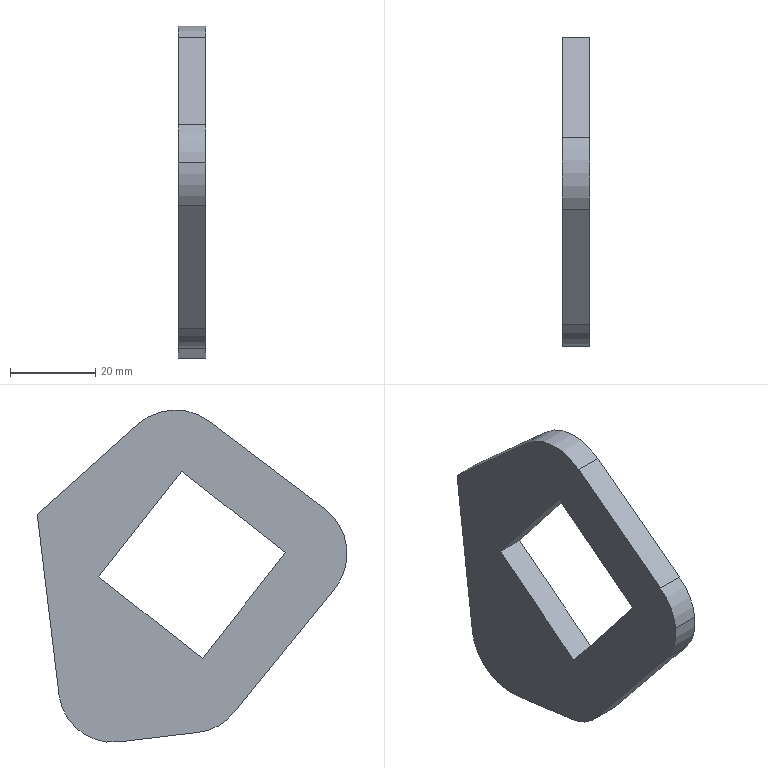Component | SolidWorks | DNR-71M20100BBEF2xx-A_500997-1_DNR-71M20100BBEF2xx-A_500995-1 | 1 solid | 16 faces | box 6.35 x 72.84 x 78.16 mm | volume 19050 mm3 | plane 11 | cylinder 5 | commonest cylinder face diameters 26.591 x3 25.4 x2
build123d program:
from build123d import *

# Parameters (mm, degrees)
EXTRUDE1_DEPTH = 3.175
FILLET1_R      = 12.7


with BuildPart() as part:
    # Sketch1 → Extrude1 (new, symmetric)
    with BuildSketch(Plane.XY):
        with BuildLine():
            Line((-3.399, -39.116), (-34.925, -39.116))
            Line((-34.925, -39.116), (-34.925, 16.338))
            Line((-34.925, 16.338), (-8.981, 34.504))
            ThreePointArc((-8.981, 34.504), (-0.3095, 36.867), (7.884, 33.174))
            Line((7.884, 33.174), (32.321, 9.561))
            ThreePointArc((32.321, 9.561), (36.377, 0), (32.321, -9.561))
            Line((32.321, -9.561), (5.426, -35.549))
            ThreePointArc((5.426, -35.549), (1.361, -38.19), (-3.399, -39.116))
        make_face()
        Polygon((0, 22.351), (-22.352, 0), (-0.3962, -21.957), (21.956, 0.3937), align=None, mode=Mode.SUBTRACT)
    extrude(amount=EXTRUDE1_DEPTH, both=True)

    # Fillet1
    fillet1_edges = [part.edges().sort_by_distance(p)[0] for p in [
        (-34.925, -39.116, 0),
    ]]
    fillet(fillet1_edges, radius=FILLET1_R)


solid = part.part

# Placed as in the assembly
solid = solid.moved(Location((301.625, -113.427, 165.976), (83.13, -90, 0)))
STEP:
#1=COLOUR_RGB('',0.7922,0.8196,0.9333);
#2=FILL_AREA_STYLE_COLOUR('',#1);
#3=FILL_AREA_STYLE('',(#2));
#4=SURFACE_STYLE_FILL_AREA(#3);
#5=SURFACE_SIDE_STYLE('',(#4));
#6=SURFACE_STYLE_USAGE(.BOTH.,#5);
#7=PRESENTATION_STYLE_ASSIGNMENT((#6));
#8=CARTESIAN_POINT('',(12.,-5.774,6.313));
#9=VERTEX_POINT('',#8);
#10=CARTESIAN_POINT('',(12.,-5.888,6.706));
#11=VERTEX_POINT('',#10);
#12=CARTESIAN_POINT('',(12.,-5.368,6.643));
#13=DIRECTION('',(-1.,0.,0.));
#14=DIRECTION('',(0.,0.9928,-0.1196));
#15=AXIS2_PLACEMENT_3D('',#12,#13,#14);
#16=CIRCLE('',#15,0.5234);
#17=EDGE_CURVE('',#9,#11,#16,.T.);
#18=ORIENTED_EDGE('',*,*,#17,.T.);
#19=CARTESIAN_POINT('',(11.75,-5.888,6.706));
#20=VERTEX_POINT('',#19);
#21=CARTESIAN_POINT('',(12.,-5.888,6.706));
#22=DIRECTION('',(-1.,0.,0.));
#23=VECTOR('',#22,39.37);
#24=LINE('',#21,#23);
#25=EDGE_CURVE('',#11,#20,#24,.T.);
#26=ORIENTED_EDGE('',*,*,#25,.T.);
#27=CARTESIAN_POINT('',(11.75,-5.774,6.313));
#28=VERTEX_POINT('',#27);
#29=CARTESIAN_POINT('',(11.75,-5.368,6.643));
#30=DIRECTION('',(-1.,0.,0.));
#31=DIRECTION('',(0.,0.9928,-0.1196));
#32=AXIS2_PLACEMENT_3D('',#29,#30,#31);
#33=CIRCLE('',#32,0.5234);
#34=EDGE_CURVE('',#28,#20,#33,.T.);
#35=ORIENTED_EDGE('',*,*,#34,.F.);
#36=CARTESIAN_POINT('',(12.,-5.774,6.313));
#37=DIRECTION('',(-1.,0.,0.));
#38=VECTOR('',#37,39.37);
#39=LINE('',#36,#38);
#40=EDGE_CURVE('',#9,#28,#39,.T.);
#41=ORIENTED_EDGE('',*,*,#40,.F.);
#42=EDGE_LOOP('',(#18,#26,#35,#41));
#43=FACE_OUTER_BOUND('',#42,.T.);
#44=CARTESIAN_POINT('',(12.,-5.368,6.643));
#45=DIRECTION('',(-1.,0.,0.));
#46=DIRECTION('',(0.,-0.9928,0.1196));
#47=AXIS2_PLACEMENT_3D('',#44,#45,#46);
#48=CYLINDRICAL_SURFACE('',#47,0.5234);
#49=ADVANCED_FACE('',(#43),#48,.T.);
#50=CARTESIAN_POINT('',(12.,-3.024,7.009));
#51=VERTEX_POINT('',#50);
#52=CARTESIAN_POINT('',(12.,-3.225,5.337));
#53=VERTEX_POINT('',#52);
#54=CARTESIAN_POINT('',(12.,-3.285,4.841));
#55=DIRECTION('',(-0.,-0.1196,-0.9928));
#56=VECTOR('',#55,39.37);
#57=LINE('',#54,#56);
#58=EDGE_CURVE('',#51,#53,#57,.T.);
#59=ORIENTED_EDGE('',*,*,#58,.T.);
#60=CARTESIAN_POINT('',(11.75,-3.225,5.337));
#61=VERTEX_POINT('',#60);
#62=CARTESIAN_POINT('',(12.,-3.225,5.337));
#63=DIRECTION('',(-1.,0.,0.));
#64=VECTOR('',#63,39.37);
#65=LINE('',#62,#64);
#66=EDGE_CURVE('',#53,#61,#65,.T.);
#67=ORIENTED_EDGE('',*,*,#66,.T.);
#68=CARTESIAN_POINT('',(11.75,-3.024,7.009));
#69=VERTEX_POINT('',#68);
#70=CARTESIAN_POINT('',(11.75,-3.285,4.841));
#71=DIRECTION('',(-0.,-0.1196,-0.9928));
#72=VECTOR('',#71,39.37);
#73=LINE('',#70,#72);
#74=EDGE_CURVE('',#69,#61,#73,.T.);
#75=ORIENTED_EDGE('',*,*,#74,.F.);
#76=CARTESIAN_POINT('',(12.,-3.024,7.009));
#77=DIRECTION('',(-1.,0.,0.));
#78=VECTOR('',#77,39.37);
#79=LINE('',#76,#78);
#80=EDGE_CURVE('',#51,#69,#79,.T.);
#81=ORIENTED_EDGE('',*,*,#80,.F.);
#82=EDGE_LOOP('',(#59,#67,#75,#81));
#83=FACE_OUTER_BOUND('',#82,.T.);
#84=CARTESIAN_POINT('',(12.,-3.285,4.841));
#85=DIRECTION('',(-0.,0.9928,-0.1196));
#86=DIRECTION('',(-1.,0.,0.));
#87=AXIS2_PLACEMENT_3D('',#84,#85,#86);
#88=PLANE('',#87);
#89=ADVANCED_FACE('',(#83),#88,.T.);
#90=CARTESIAN_POINT('',(11.75,-3.952,7.841));
#91=VERTEX_POINT('',#90);
#92=CARTESIAN_POINT('',(11.75,-3.024,7.009));
#93=DIRECTION('',(-0.,0.7447,-0.6674));
#94=VECTOR('',#93,39.37);
#95=LINE('',#92,#94);
#96=EDGE_CURVE('',#91,#69,#95,.T.);
#97=ORIENTED_EDGE('',*,*,#96,.F.);
#98=CARTESIAN_POINT('',(12.,-3.952,7.841));
#99=VERTEX_POINT('',#98);
#100=CARTESIAN_POINT('',(12.,-3.952,7.841));
#101=DIRECTION('',(-1.,0.,0.));
#102=VECTOR('',#101,39.37);
#103=LINE('',#100,#102);
#104=EDGE_CURVE('',#99,#91,#103,.T.);
#105=ORIENTED_EDGE('',*,*,#104,.F.);
#106=CARTESIAN_POINT('',(12.,-3.024,7.009));
#107=DIRECTION('',(-0.,0.7447,-0.6674));
#108=VECTOR('',#107,39.37);
#109=LINE('',#106,#108);
#110=EDGE_CURVE('',#99,#51,#109,.T.);
#111=ORIENTED_EDGE('',*,*,#110,.T.);
#112=ORIENTED_EDGE('',*,*,#80,.T.);
#113=EDGE_LOOP('',(#97,#105,#111,#112));
#114=FACE_OUTER_BOUND('',#113,.T.);
#115=CARTESIAN_POINT('',(12.,-3.024,7.009));
#116=DIRECTION('',(0.,0.6674,0.7447));
#117=DIRECTION('',(-0.,0.7447,-0.6674));
#118=AXIS2_PLACEMENT_3D('',#115,#116,#117);
#119=PLANE('',#118);
#120=ADVANCED_FACE('',(#114),#119,.T.);
#121=CARTESIAN_POINT('',(11.75,-4.618,7.868));
#122=VERTEX_POINT('',#121);
#123=CARTESIAN_POINT('',(11.75,-4.301,7.451));
#124=DIRECTION('',(-1.,0.,0.));
#125=DIRECTION('',(0.,-0.9928,0.1196));
#126=AXIS2_PLACEMENT_3D('',#123,#124,#125);
#127=CIRCLE('',#126,0.5234);
#128=EDGE_CURVE('',#122,#91,#127,.T.);
#129=ORIENTED_EDGE('',*,*,#128,.F.);
#130=CARTESIAN_POINT('',(12.,-4.618,7.868));
#131=VERTEX_POINT('',#130);
#132=CARTESIAN_POINT('',(12.,-4.618,7.868));
#133=DIRECTION('',(-1.,0.,0.));
#134=VECTOR('',#133,39.37);
#135=LINE('',#132,#134);
#136=EDGE_CURVE('',#131,#122,#135,.T.);
#137=ORIENTED_EDGE('',*,*,#136,.F.);
#138=CARTESIAN_POINT('',(12.,-4.301,7.451));
#139=DIRECTION('',(-1.,0.,0.));
#140=DIRECTION('',(0.,-0.9928,0.1196));
#141=AXIS2_PLACEMENT_3D('',#138,#139,#140);
#142=CIRCLE('',#141,0.5234);
#143=EDGE_CURVE('',#131,#99,#142,.T.);
#144=ORIENTED_EDGE('',*,*,#143,.T.);
#145=ORIENTED_EDGE('',*,*,#104,.T.);
#146=EDGE_LOOP('',(#129,#137,#144,#145));
#147=FACE_OUTER_BOUND('',#146,.T.);
#148=CARTESIAN_POINT('',(12.,-4.301,7.451));
#149=DIRECTION('',(-1.,0.,0.));
#150=DIRECTION('',(0.,-0.9928,0.1196));
#151=AXIS2_PLACEMENT_3D('',#148,#149,#150);
#152=CYLINDRICAL_SURFACE('',#151,0.5234);
#153=ADVANCED_FACE('',(#147),#152,.T.);
#154=CARTESIAN_POINT('',(11.75,-5.684,7.06));
#155=VERTEX_POINT('',#154);
#156=CARTESIAN_POINT('',(11.75,-4.618,7.868));
#157=DIRECTION('',(0.,0.7971,0.6039));
#158=VECTOR('',#157,39.37);
#159=LINE('',#156,#158);
#160=EDGE_CURVE('',#155,#122,#159,.T.);
#161=ORIENTED_EDGE('',*,*,#160,.F.);
#162=CARTESIAN_POINT('',(12.,-5.684,7.06));
#163=VERTEX_POINT('',#162);
#164=CARTESIAN_POINT('',(12.,-5.684,7.06));
#165=DIRECTION('',(-1.,0.,0.));
#166=VECTOR('',#165,39.37);
#167=LINE('',#164,#166);
#168=EDGE_CURVE('',#163,#155,#167,.T.);
#169=ORIENTED_EDGE('',*,*,#168,.F.);
#170=CARTESIAN_POINT('',(12.,-4.618,7.868));
#171=DIRECTION('',(0.,0.7971,0.6039));
#172=VECTOR('',#171,39.37);
#173=LINE('',#170,#172);
#174=EDGE_CURVE('',#163,#131,#173,.T.);
#175=ORIENTED_EDGE('',*,*,#174,.T.);
#176=ORIENTED_EDGE('',*,*,#136,.T.);
#177=EDGE_LOOP('',(#161,#169,#175,#176));
#178=FACE_OUTER_BOUND('',#177,.T.);
#179=CARTESIAN_POINT('',(12.,-4.618,7.868));
#180=DIRECTION('',(0.,-0.6039,0.7971));
#181=DIRECTION('',(0.,0.7971,0.6039));
#182=AXIS2_PLACEMENT_3D('',#179,#180,#181);
#183=PLANE('',#182);
#184=ADVANCED_FACE('',(#178),#183,.T.);
#185=ORIENTED_EDGE('',*,*,#25,.F.);
#186=CARTESIAN_POINT('',(12.,-5.368,6.643));
#187=DIRECTION('',(-1.,0.,0.));
#188=DIRECTION('',(0.,0.9928,-0.1196));
#189=AXIS2_PLACEMENT_3D('',#186,#187,#188);
#190=CIRCLE('',#189,0.5234);
#191=EDGE_CURVE('',#11,#163,#190,.T.);
#192=ORIENTED_EDGE('',*,*,#191,.T.);
#193=ORIENTED_EDGE('',*,*,#168,.T.);
#194=CARTESIAN_POINT('',(11.75,-5.368,6.643));
#195=DIRECTION('',(-1.,0.,0.));
#196=DIRECTION('',(0.,0.9928,-0.1196));
#197=AXIS2_PLACEMENT_3D('',#194,#195,#196);
#198=CIRCLE('',#197,0.5234);
#199=EDGE_CURVE('',#20,#155,#198,.T.);
#200=ORIENTED_EDGE('',*,*,#199,.F.);
#201=EDGE_LOOP('',(#185,#192,#193,#200));
#202=FACE_OUTER_BOUND('',#201,.T.);
#203=CARTESIAN_POINT('',(12.,-5.368,6.643));
#204=DIRECTION('',(-1.,0.,0.));
#205=DIRECTION('',(0.,-0.9928,0.1196));
#206=AXIS2_PLACEMENT_3D('',#203,#204,#205);
#207=CYLINDRICAL_SURFACE('',#206,0.5234);
#208=ADVANCED_FACE('',(#202),#207,.T.);
#209=CARTESIAN_POINT('',(11.75,-4.845,5.171));
#210=VERTEX_POINT('',#209);
#211=CARTESIAN_POINT('',(11.75,-5.774,6.313));
#212=DIRECTION('',(0.,-0.6308,0.7759));
#213=VECTOR('',#212,39.37);
#214=LINE('',#211,#213);
#215=EDGE_CURVE('',#210,#28,#214,.T.);
#216=ORIENTED_EDGE('',*,*,#215,.F.);
#217=CARTESIAN_POINT('',(12.,-4.845,5.171));
#218=VERTEX_POINT('',#217);
#219=CARTESIAN_POINT('',(12.,-4.845,5.171));
#220=DIRECTION('',(-1.,0.,0.));
#221=VECTOR('',#220,39.37);
#222=LINE('',#219,#221);
#223=EDGE_CURVE('',#218,#210,#222,.T.);
#224=ORIENTED_EDGE('',*,*,#223,.F.);
#225=CARTESIAN_POINT('',(12.,-5.774,6.313));
#226=DIRECTION('',(0.,-0.6308,0.7759));
#227=VECTOR('',#226,39.37);
#228=LINE('',#225,#227);
#229=EDGE_CURVE('',#218,#9,#228,.T.);
#230=ORIENTED_EDGE('',*,*,#229,.T.);
#231=ORIENTED_EDGE('',*,*,#40,.T.);
#232=EDGE_LOOP('',(#216,#224,#230,#231));
#233=FACE_OUTER_BOUND('',#232,.T.);
#234=CARTESIAN_POINT('',(12.,-5.774,6.313));
#235=DIRECTION('',(-0.,-0.7759,-0.6308));
#236=DIRECTION('',(0.,-0.6308,0.7759));
#237=AXIS2_PLACEMENT_3D('',#234,#235,#236);
#238=PLANE('',#237);
#239=ADVANCED_FACE('',(#233),#238,.T.);
#240=CARTESIAN_POINT('',(11.75,-4.517,4.99));
#241=VERTEX_POINT('',#240);
#242=CARTESIAN_POINT('',(11.75,-4.457,5.486));
#243=DIRECTION('',(-1.,0.,0.));
#244=DIRECTION('',(0.,0.9928,-0.1196));
#245=AXIS2_PLACEMENT_3D('',#242,#243,#244);
#246=CIRCLE('',#245,0.5);
#247=EDGE_CURVE('',#241,#210,#246,.T.);
#248=ORIENTED_EDGE('',*,*,#247,.F.);
#249=CARTESIAN_POINT('',(12.,-4.517,4.99));
#250=VERTEX_POINT('',#249);
#251=CARTESIAN_POINT('',(12.,-4.517,4.99));
#252=DIRECTION('',(-1.,0.,0.));
#253=VECTOR('',#252,39.37);
#254=LINE('',#251,#253);
#255=EDGE_CURVE('',#250,#241,#254,.T.);
#256=ORIENTED_EDGE('',*,*,#255,.F.);
#257=CARTESIAN_POINT('',(12.,-4.457,5.486));
#258=DIRECTION('',(-1.,0.,0.));
#259=DIRECTION('',(0.,0.9928,-0.1196));
#260=AXIS2_PLACEMENT_3D('',#257,#258,#259);
#261=CIRCLE('',#260,0.5);
#262=EDGE_CURVE('',#250,#218,#261,.T.);
#263=ORIENTED_EDGE('',*,*,#262,.T.);
#264=ORIENTED_EDGE('',*,*,#223,.T.);
#265=EDGE_LOOP('',(#248,#256,#263,#264));
#266=FACE_OUTER_BOUND('',#265,.T.);
#267=CARTESIAN_POINT('',(12.,-4.457,5.486));
#268=DIRECTION('',(-1.,0.,0.));
#269=DIRECTION('',(0.,-0.9928,0.1196));
#270=AXIS2_PLACEMENT_3D('',#267,#268,#269);
#271=CYLINDRICAL_SURFACE('',#270,0.5);
#272=ADVANCED_FACE('',(#266),#271,.T.);
#273=CARTESIAN_POINT('',(11.75,-3.781,4.901));
#274=VERTEX_POINT('',#273);
#275=CARTESIAN_POINT('',(11.75,-4.517,4.99));
#276=DIRECTION('',(0.,-0.9928,0.1196));
#277=VECTOR('',#276,39.37);
#278=LINE('',#275,#277);
#279=EDGE_CURVE('',#274,#241,#278,.T.);
#280=ORIENTED_EDGE('',*,*,#279,.F.);
#281=CARTESIAN_POINT('',(12.,-3.781,4.901));
#282=VERTEX_POINT('',#281);
#283=CARTESIAN_POINT('',(12.,-3.781,4.901));
#284=DIRECTION('',(1.,-0.,-0.));
#285=VECTOR('',#284,39.37);
#286=LINE('',#283,#285);
#287=EDGE_CURVE('',#274,#282,#286,.T.);
#288=ORIENTED_EDGE('',*,*,#287,.T.);
#289=CARTESIAN_POINT('',(12.,-4.517,4.99));
#290=DIRECTION('',(0.,-0.9928,0.1196));
#291=VECTOR('',#290,39.37);
#292=LINE('',#289,#291);
#293=EDGE_CURVE('',#282,#250,#292,.T.);
#294=ORIENTED_EDGE('',*,*,#293,.T.);
#295=ORIENTED_EDGE('',*,*,#255,.T.);
#296=EDGE_LOOP('',(#280,#288,#294,#295));
#297=FACE_OUTER_BOUND('',#296,.T.);
#298=CARTESIAN_POINT('',(12.,-4.517,4.99));
#299=DIRECTION('',(-0.,-0.1196,-0.9928));
#300=DIRECTION('',(0.,-0.9928,0.1196));
#301=AXIS2_PLACEMENT_3D('',#298,#299,#300);
#302=PLANE('',#301);
#303=ADVANCED_FACE('',(#297),#302,.T.);
#304=CARTESIAN_POINT('',(12.,-4.554,5.674));
#305=VERTEX_POINT('',#304);
#306=CARTESIAN_POINT('',(12.,-5.322,6.653));
#307=VERTEX_POINT('',#306);
#308=CARTESIAN_POINT('',(12.,-4.554,5.674));
#309=DIRECTION('',(0.,-0.6175,0.7866));
#310=VECTOR('',#309,39.37);
#311=LINE('',#308,#310);
#312=EDGE_CURVE('',#305,#307,#311,.T.);
#313=ORIENTED_EDGE('',*,*,#312,.T.);
#314=CARTESIAN_POINT('',(12.,-4.36,7.408));
#315=VERTEX_POINT('',#314);
#316=CARTESIAN_POINT('',(12.,-5.322,6.653));
#317=DIRECTION('',(0.,0.7866,0.6175));
#318=VECTOR('',#317,39.37);
#319=LINE('',#316,#318);
#320=EDGE_CURVE('',#307,#315,#319,.T.);
#321=ORIENTED_EDGE('',*,*,#320,.T.);
#322=CARTESIAN_POINT('',(12.,-3.592,6.429));
#323=VERTEX_POINT('',#322);
#324=CARTESIAN_POINT('',(12.,-4.36,7.408));
#325=DIRECTION('',(-0.,0.6175,-0.7866));
#326=VECTOR('',#325,39.37);
#327=LINE('',#324,#326);
#328=EDGE_CURVE('',#315,#323,#327,.T.);
#329=ORIENTED_EDGE('',*,*,#328,.T.);
#330=CARTESIAN_POINT('',(12.,-3.592,6.429));
#331=DIRECTION('',(-0.,-0.7866,-0.6175));
#332=VECTOR('',#331,39.37);
#333=LINE('',#330,#332);
#334=EDGE_CURVE('',#323,#305,#333,.T.);
#335=ORIENTED_EDGE('',*,*,#334,.T.);
#336=EDGE_LOOP('',(#313,#321,#329,#335));
#337=FACE_BOUND('',#336,.T.);
#338=ORIENTED_EDGE('',*,*,#293,.F.);
#339=CARTESIAN_POINT('',(12.,-3.721,5.397));
#340=DIRECTION('',(1.,-0.,-0.));
#341=DIRECTION('',(0.,-0.9928,0.1196));
#342=AXIS2_PLACEMENT_3D('',#339,#340,#341);
#343=CIRCLE('',#342,0.5);
#344=EDGE_CURVE('',#282,#53,#343,.T.);
#345=ORIENTED_EDGE('',*,*,#344,.T.);
#346=ORIENTED_EDGE('',*,*,#58,.F.);
#347=ORIENTED_EDGE('',*,*,#110,.F.);
#348=ORIENTED_EDGE('',*,*,#143,.F.);
#349=ORIENTED_EDGE('',*,*,#174,.F.);
#350=ORIENTED_EDGE('',*,*,#191,.F.);
#351=ORIENTED_EDGE('',*,*,#17,.F.);
#352=ORIENTED_EDGE('',*,*,#229,.F.);
#353=ORIENTED_EDGE('',*,*,#262,.F.);
#354=EDGE_LOOP('',(#338,#345,#346,#347,#348,#349,#350,#351,#352,#353));
#355=FACE_OUTER_BOUND('',#354,.T.);
#356=CARTESIAN_POINT('',(12.,-4.301,7.451));
#357=DIRECTION('',(-1.,0.,0.));
#358=DIRECTION('',(0.,-0.9928,0.1196));
#359=AXIS2_PLACEMENT_3D('',#356,#357,#358);
#360=PLANE('',#359);
#361=ADVANCED_FACE('',(#337,#355),#360,.F.);
#362=CARTESIAN_POINT('',(11.75,-5.322,6.653));
#363=VERTEX_POINT('',#362);
#364=CARTESIAN_POINT('',(11.75,-4.36,7.408));
#365=VERTEX_POINT('',#364);
#366=CARTESIAN_POINT('',(11.75,-5.322,6.653));
#367=DIRECTION('',(0.,0.7866,0.6175));
#368=VECTOR('',#367,39.37);
#369=LINE('',#366,#368);
#370=EDGE_CURVE('',#363,#365,#369,.T.);
#371=ORIENTED_EDGE('',*,*,#370,.F.);
#372=CARTESIAN_POINT('',(11.75,-4.554,5.674));
#373=VERTEX_POINT('',#372);
#374=CARTESIAN_POINT('',(11.75,-4.554,5.674));
#375=DIRECTION('',(0.,-0.6175,0.7866));
#376=VECTOR('',#375,39.37);
#377=LINE('',#374,#376);
#378=EDGE_CURVE('',#373,#363,#377,.T.);
#379=ORIENTED_EDGE('',*,*,#378,.F.);
#380=CARTESIAN_POINT('',(11.75,-3.592,6.429));
#381=VERTEX_POINT('',#380);
#382=CARTESIAN_POINT('',(11.75,-3.592,6.429));
#383=DIRECTION('',(-0.,-0.7866,-0.6175));
#384=VECTOR('',#383,39.37);
#385=LINE('',#382,#384);
#386=EDGE_CURVE('',#381,#373,#385,.T.);
#387=ORIENTED_EDGE('',*,*,#386,.F.);
#388=CARTESIAN_POINT('',(11.75,-4.36,7.408));
#389=DIRECTION('',(-0.,0.6175,-0.7866));
#390=VECTOR('',#389,39.37);
#391=LINE('',#388,#390);
#392=EDGE_CURVE('',#365,#381,#391,.T.);
#393=ORIENTED_EDGE('',*,*,#392,.F.);
#394=EDGE_LOOP('',(#371,#379,#387,#393));
#395=FACE_BOUND('',#394,.T.);
#396=ORIENTED_EDGE('',*,*,#74,.T.);
#397=CARTESIAN_POINT('',(11.75,-3.721,5.397));
#398=DIRECTION('',(-1.,0.,0.));
#399=DIRECTION('',(0.,-0.9928,0.1196));
#400=AXIS2_PLACEMENT_3D('',#397,#398,#399);
#401=CIRCLE('',#400,0.5);
#402=EDGE_CURVE('',#61,#274,#401,.T.);
#403=ORIENTED_EDGE('',*,*,#402,.T.);
#404=ORIENTED_EDGE('',*,*,#279,.T.);
#405=ORIENTED_EDGE('',*,*,#247,.T.);
#406=ORIENTED_EDGE('',*,*,#215,.T.);
#407=ORIENTED_EDGE('',*,*,#34,.T.);
#408=ORIENTED_EDGE('',*,*,#199,.T.);
#409=ORIENTED_EDGE('',*,*,#160,.T.);
#410=ORIENTED_EDGE('',*,*,#128,.T.);
#411=ORIENTED_EDGE('',*,*,#96,.T.);
#412=EDGE_LOOP('',(#396,#403,#404,#405,#406,#407,#408,#409,#410,#411));
#413=FACE_OUTER_BOUND('',#412,.T.);
#414=CARTESIAN_POINT('',(11.75,-4.301,7.451));
#415=DIRECTION('',(-1.,0.,0.));
#416=DIRECTION('',(0.,-0.9928,0.1196));
#417=AXIS2_PLACEMENT_3D('',#414,#415,#416);
#418=PLANE('',#417);
#419=ADVANCED_FACE('',(#395,#413),#418,.T.);
#420=ORIENTED_EDGE('',*,*,#370,.T.);
#421=CARTESIAN_POINT('',(12.,-4.36,7.408));
#422=DIRECTION('',(-1.,0.,0.));
#423=VECTOR('',#422,39.37);
#424=LINE('',#421,#423);
#425=EDGE_CURVE('',#315,#365,#424,.T.);
#426=ORIENTED_EDGE('',*,*,#425,.F.);
#427=ORIENTED_EDGE('',*,*,#320,.F.);
#428=CARTESIAN_POINT('',(12.,-5.322,6.653));
#429=DIRECTION('',(-1.,0.,0.));
#430=VECTOR('',#429,39.37);
#431=LINE('',#428,#430);
#432=EDGE_CURVE('',#307,#363,#431,.T.);
#433=ORIENTED_EDGE('',*,*,#432,.T.);
#434=EDGE_LOOP('',(#420,#426,#427,#433));
#435=FACE_OUTER_BOUND('',#434,.T.);
#436=CARTESIAN_POINT('',(12.,-5.322,6.653));
#437=DIRECTION('',(0.,-0.6175,0.7866));
#438=DIRECTION('',(0.,0.7866,0.6175));
#439=AXIS2_PLACEMENT_3D('',#436,#437,#438);
#440=PLANE('',#439);
#441=ADVANCED_FACE('',(#435),#440,.F.);
#442=ORIENTED_EDGE('',*,*,#378,.T.);
#443=ORIENTED_EDGE('',*,*,#432,.F.);
#444=ORIENTED_EDGE('',*,*,#312,.F.);
#445=CARTESIAN_POINT('',(12.,-4.554,5.674));
#446=DIRECTION('',(-1.,0.,0.));
#447=VECTOR('',#446,39.37);
#448=LINE('',#445,#447);
#449=EDGE_CURVE('',#305,#373,#448,.T.);
#450=ORIENTED_EDGE('',*,*,#449,.T.);
#451=EDGE_LOOP('',(#442,#443,#444,#450));
#452=FACE_OUTER_BOUND('',#451,.T.);
#453=CARTESIAN_POINT('',(12.,-4.554,5.674));
#454=DIRECTION('',(-0.,-0.7866,-0.6175));
#455=DIRECTION('',(0.,-0.6175,0.7866));
#456=AXIS2_PLACEMENT_3D('',#453,#454,#455);
#457=PLANE('',#456);
#458=ADVANCED_FACE('',(#452),#457,.F.);
#459=ORIENTED_EDGE('',*,*,#386,.T.);
#460=ORIENTED_EDGE('',*,*,#449,.F.);
#461=ORIENTED_EDGE('',*,*,#334,.F.);
#462=CARTESIAN_POINT('',(12.,-3.592,6.429));
#463=DIRECTION('',(-1.,0.,0.));
#464=VECTOR('',#463,39.37);
#465=LINE('',#462,#464);
#466=EDGE_CURVE('',#323,#381,#465,.T.);
#467=ORIENTED_EDGE('',*,*,#466,.T.);
#468=EDGE_LOOP('',(#459,#460,#461,#467));
#469=FACE_OUTER_BOUND('',#468,.T.);
#470=CARTESIAN_POINT('',(12.,-3.592,6.429));
#471=DIRECTION('',(-0.,0.6175,-0.7866));
#472=DIRECTION('',(-0.,-0.7866,-0.6175));
#473=AXIS2_PLACEMENT_3D('',#470,#471,#472);
#474=PLANE('',#473);
#475=ADVANCED_FACE('',(#469),#474,.F.);
#476=ORIENTED_EDGE('',*,*,#392,.T.);
#477=ORIENTED_EDGE('',*,*,#466,.F.);
#478=ORIENTED_EDGE('',*,*,#328,.F.);
#479=ORIENTED_EDGE('',*,*,#425,.T.);
#480=EDGE_LOOP('',(#476,#477,#478,#479));
#481=FACE_OUTER_BOUND('',#480,.T.);
#482=CARTESIAN_POINT('',(12.,-4.36,7.408));
#483=DIRECTION('',(0.,0.7866,0.6175));
#484=DIRECTION('',(-0.,0.6175,-0.7866));
#485=AXIS2_PLACEMENT_3D('',#482,#483,#484);
#486=PLANE('',#485);
#487=ADVANCED_FACE('',(#481),#486,.F.);
#488=ORIENTED_EDGE('',*,*,#344,.F.);
#489=ORIENTED_EDGE('',*,*,#287,.F.);
#490=ORIENTED_EDGE('',*,*,#402,.F.);
#491=ORIENTED_EDGE('',*,*,#66,.F.);
#492=EDGE_LOOP('',(#488,#489,#490,#491));
#493=FACE_OUTER_BOUND('',#492,.T.);
#494=CARTESIAN_POINT('',(12.,-3.721,5.397));
#495=DIRECTION('',(-1.,0.,0.));
#496=DIRECTION('',(0.,-0.9928,0.1196));
#497=AXIS2_PLACEMENT_3D('',#494,#495,#496);
#498=CYLINDRICAL_SURFACE('',#497,0.5);
#499=ADVANCED_FACE('',(#493),#498,.T.);
#500=CLOSED_SHELL('',(#49,#89,#120,#153,#184,#208,#239,#272,#303,#361,#419,#441,#458,#475,#487,#499));
#501=MANIFOLD_SOLID_BREP('',#500);
#502=STYLED_ITEM('',(#7),#501);
#503=(LENGTH_UNIT()NAMED_UNIT(*)SI_UNIT($,.METRE.));
#504=LENGTH_MEASURE_WITH_UNIT(LENGTH_MEASURE(0.0254),#503);
#505=DIMENSIONAL_EXPONENTS(1.,0.,0.,0.,0.,0.,0.);
#506=(CONVERSION_BASED_UNIT('',#504)LENGTH_UNIT()NAMED_UNIT(#505));
#507=UNCERTAINTY_MEASURE_WITH_UNIT(LENGTH_MEASURE(0.00001),#506,'','');
#508=(NAMED_UNIT(*)PLANE_ANGLE_UNIT()SI_UNIT($,.RADIAN.));
#509=(NAMED_UNIT(*)SI_UNIT($,.STERADIAN.)SOLID_ANGLE_UNIT());
#510=(GEOMETRIC_REPRESENTATION_CONTEXT(3)GLOBAL_UNCERTAINTY_ASSIGNED_CONTEXT((#507))GLOBAL_UNIT_ASSIGNED_CONTEXT((#506,#508,#509))REPRESENTATION_CONTEXT('',''));
#511=MECHANICAL_DESIGN_GEOMETRIC_PRESENTATION_REPRESENTATION('',(#502),#510);
#512=CARTESIAN_POINT('',(0.,0.,0.));
#513=DIRECTION('',(0.,0.,1.));
#514=DIRECTION('',(1.,0.,0.));
#515=AXIS2_PLACEMENT_3D('',#512,#513,#514);
#516=(LENGTH_UNIT()NAMED_UNIT(*)SI_UNIT($,.METRE.));
#517=LENGTH_MEASURE_WITH_UNIT(LENGTH_MEASURE(0.0254),#516);
#518=DIMENSIONAL_EXPONENTS(1.,0.,0.,0.,0.,0.,0.);
#519=(CONVERSION_BASED_UNIT('',#517)LENGTH_UNIT()NAMED_UNIT(#518));
#520=UNCERTAINTY_MEASURE_WITH_UNIT(LENGTH_MEASURE(0.00001),#519,'','');
#521=(NAMED_UNIT(*)PLANE_ANGLE_UNIT()SI_UNIT($,.RADIAN.));
#522=(NAMED_UNIT(*)SI_UNIT($,.STERADIAN.)SOLID_ANGLE_UNIT());
#523=(GEOMETRIC_REPRESENTATION_CONTEXT(3)GLOBAL_UNCERTAINTY_ASSIGNED_CONTEXT((#520))GLOBAL_UNIT_ASSIGNED_CONTEXT((#519,#521,#522))REPRESENTATION_CONTEXT('',''));
#524=ADVANCED_BREP_SHAPE_REPRESENTATION('',(#501,#515),#523);
#525=PRESENTATION_LAYER_ASSIGNMENT('','',(#502));